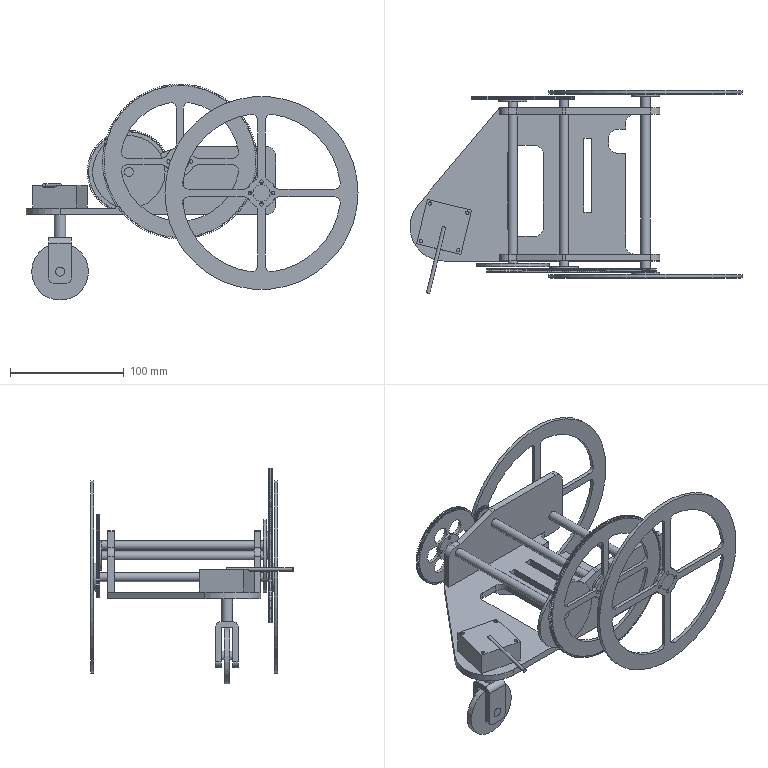Assembly | NX | mm | 16 component files | 16 solids | 2718 faces | box 292.39 x 178.71 x 190.14 mm | volume 370124 mm3 | other 2025 | cylinder 578 | plane 115 | commonest cylinder face diameters 133.5 x225 70.5 x120 16.5 x60 10 x55 3 x33 8 x20 25 x16 15 x16
Bill of materials:
unnamed part 1 | 1 |  | Clevis-style fork body: a rectangular block with rounded corners, slotted through its depth to form two parallel prongs. A coaxial cross hole runs through both prongs near the open end. A stepped cylindrical shank with two diameters sticks out from the closed end.
unnamed part 2 | 2 |  | Spur gear with straight external teeth (about 30) and a large plain central bore. Uniform face width, no hub.
unnamed part 3 | 1 |  | Thin flat circular disc with a small central through-hole, shaped like a washer or shim.
unnamed part 4 | 1 |  | Large, thin, fine-pitch spur gear with a spoked web: four straight spokes join the toothed rim to a central hub. The hub has a central bore and four small holes around it.
unnamed part 5 | 1 |  | Rectangular block with four small holes near the corners of its top face. A slender cylindrical rod lies along the top face, partly sunk into it, and extends well past one edge of the block.
unnamed part 6 | 1 |  | Thin fine-pitch spur gear with seven equal circular holes: one at the center and six arranged around it in a hexagonal pattern.
unnamed part 7 | 1 |  | Long straight cylindrical rod or tube with a circular flange at each end. Each flange has four bolt holes evenly spaced on a circle. At least one flange has a raised circular boss on its outer face.
unnamed part 8 | 1 |  | Long straight cylindrical rod with a circular flange at one end only. The flange has four bolt holes evenly spaced on a circle and a raised boss on its outer face. The other end is plain.
unnamed part 9 | 1 |  | Flat circular disc with a small central through-hole. It is noticeably thicker relative to its diameter than unnamed part 3.
unnamed part 10 | 1 |  | Bent sheet-style bracket: a flat base plate with two parallel upright side walls, forming a U-channel over part of its length. The base has one rounded tapered extension with a single hole, a rounded rectangular cutout, two narrow parallel slots, and a notched end with rounded recesses. Each side wall has an angled profile and three holes.
unnamed part 11 | 1 |  | Thick cylindrical ring or spacer with a large concentric through-bore and flat end faces.
unnamed part 12 | 2 |  | Thin flat spoked wheel plate: a smooth circular outer rim joined to a central hub by four straight spokes. The hub has a central bore and four small holes around it. There are no teeth.
unnamed part 13 | 1 |  | Long slender round rod with a thin circular flange at one end. The flange has four equally spaced round through-holes on a bolt circle, and a short, narrower raised step or boss on its outer face.
unnamed part 14 | 1 |  | Plain solid right circular cylinder with flat ends. It is about 2.5 times as long as its diameter.
Mates:
1. touch align | body 1 face | wheel_axle 1 face
2. fix | body 1 component
3. center | wheel_axle 1 face | wheel_axle 1 face | body 1 face | body 1 face
4. touch align | gear_shaft_1 1 face | body 1 face
5. distance | gear_shaft_1 1 face | wheel_axle 1 face
6. touch align | gear_shaft_2 1 face | body 1 face
7. distance | gear_shaft_2 1 face | gear_shaft_1 1 face
8. touch align | wheel 2 face | wheel_axle 1 face
9. touch align | wheel 2 face | wheel_axle 1 face
10. touch align | wheel 1 face | wheel_axle 1 face
11. touch align | wheel 1 face | wheel_axle 1 face
12. touch align | wheel 1 face | wheel_axle 1 face
13. touch align | 30_gear 2 face | wheel_axle 1 face
14. touch align | 30_gear 2 face | wheel_axle 1 face
15. touch align | 225_gear 1 face | gear_shaft_1 1 face
16. touch align | 225_gear 1 face | gear_shaft_1 1 face
17. touch align | 30_gear 1 face | gear_shaft_1 1 face
18. touch align | 30_gear 1 face | gear_shaft_1 1 face
19. touch align | 120_gear 1 face | gear_shaft_2 1 face
20. touch align | 120_gear 1 face | gear_shaft_2 1 face
21. touch align | base_circle 1 face | gear_shaft_2 1 face
22. touch align | base_circle 1 face | gear_shaft_2 1 face
23. touch align | front_wheel_support 1 face | body 1 face
24. touch align | front_wheel_support 1 face | body 1 face
25. touch align | front_wheel 1 face | front_wheel_support 1 face
26. center | front_wheel 1 face | front_wheel 1 face | front_wheel_support 1 face | front_wheel_support 1 face
27. touch align | front_wheel_axle 1 face | front_wheel_support 1 face
28. touch align | front_wheel_axle 1 face | front_wheel_support 1 face
29. touch align | flange 1 face | front_wheel_support 1 face
30. touch align | body 1 face | flange 1 face
31. touch align | block 1 face | flange 1 face
32. touch align | block 1 face | body 1 face